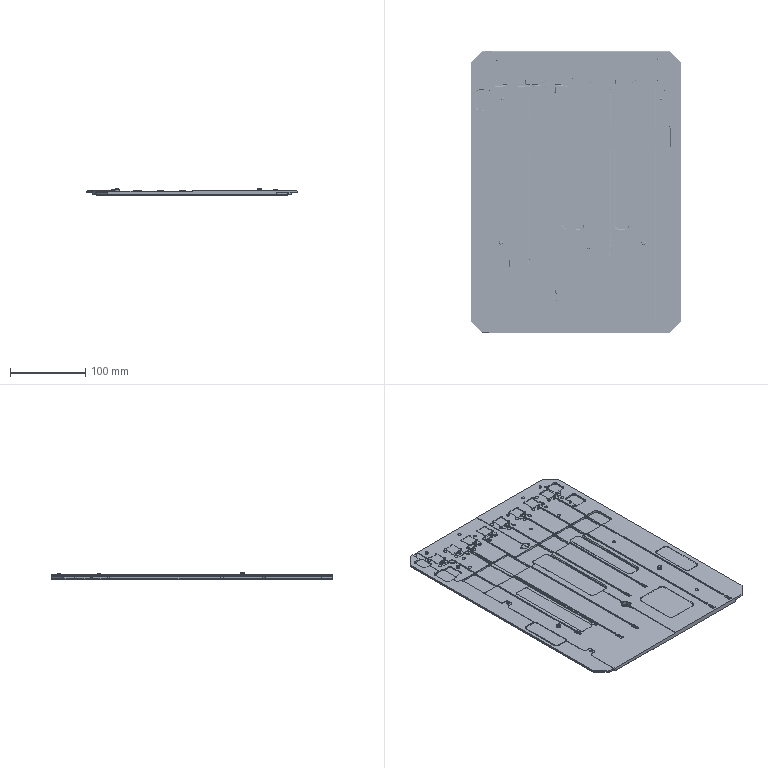CAM job | Mastercam | mm | 58 operations | part box 290 x 382 x 9.09
1. Facing | 1 - 80 面铣
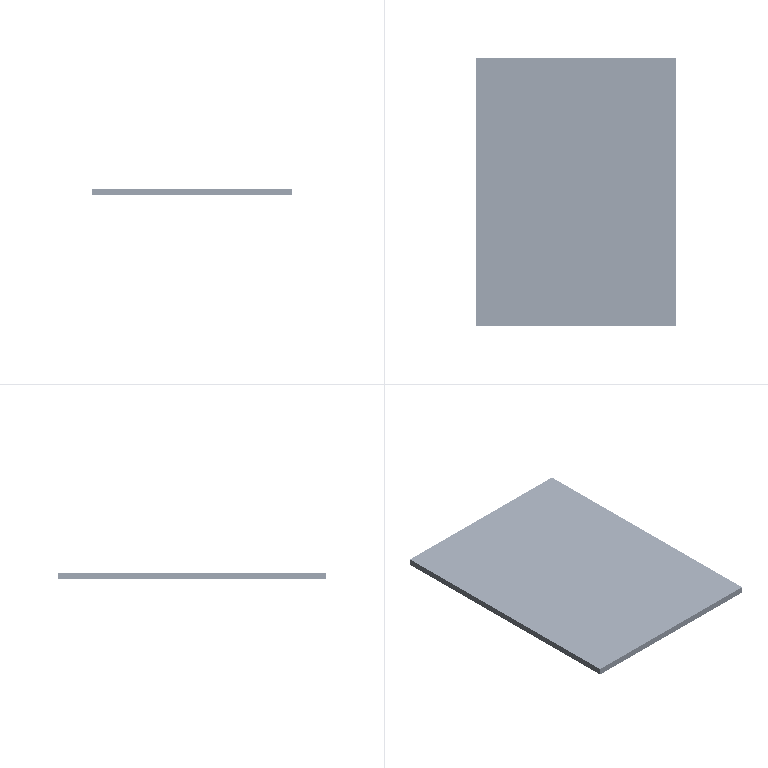2. Facing | 1 - 80 面铣
3. Contour (Ramp) | 9 - 10C 平底刀
4. Contour (2D) | 9 - 10C 平底刀
5. Contour (Ramp) | 6 - 6 平底刀
6. Contour (Remachining) | 22 - 3 平铣刀
7. Contour (Remachining) | 17 - 2 平铣刀
8. Drill/Counterbore | 2 - 4定位倒角
9. Peck Drill | 14 - 2.5 钻头
10. Peck Drill | 13 - 1.2 钻头
11. Peck Drill | 18 - 1.5 钻头
12. Peck Drill | 19 - 2 钻头
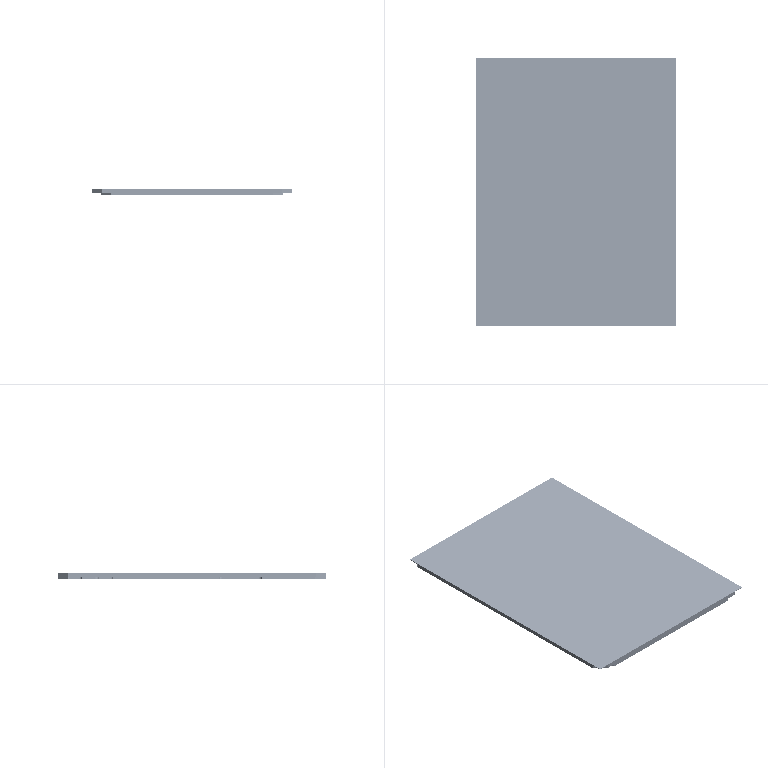13. Helix Bore | 22 - 3 平铣刀
14. Helix Bore | 22 - 3 平铣刀
15. Helix Bore | 6 - 6 平底刀
16. Surface Rough Pocket | 4 - 2-R0.5 圆鼻铣刀
17. 3D High Speed (Waterline) | 4 - 2-R0.5 圆鼻铣刀
18. Contour (Ramp) | 17 - 2 平铣刀
19. Contour (2D) | 17 - 2 平铣刀
20. Contour (Remachining) | 21 - 1 平铣刀
21. Contour (2D) | 10 - 10J 平底刀
22. Contour (2D) | 10 - 10J 平底刀
23. Contour (2D) | 22 - 3 平铣刀
24. Model Chamfer | 2 - 4定位倒角
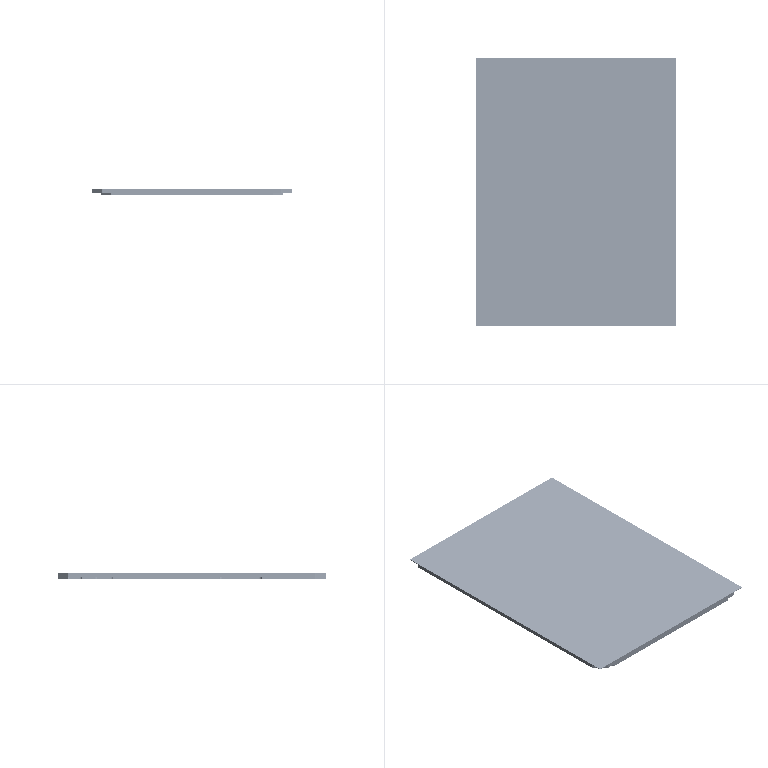25. Model Chamfer | 2 - 4定位倒角
26. Model Chamfer | 2 - 4定位倒角
27. Chamfer Drill | 2 - 4定位倒角
28. Circle Mill | 6 - 6 平底刀
29. Contour (Ramp) | 9 - 10C 平底刀
30. Surface Rough Pocket | 9 - 10C 平底刀
31. 挖槽策略 下午 09:55 | 6 - 6 平底刀
32. 挖槽策略 下午 09:55 | 7 - 4 平底刀
33. 3D High Speed (Waterline) | 6 - 6 平底刀
34. 3D High Speed (Horizontal) | 6 - 6 平底刀
35. Contour (2D) | 7 - 4 平底刀
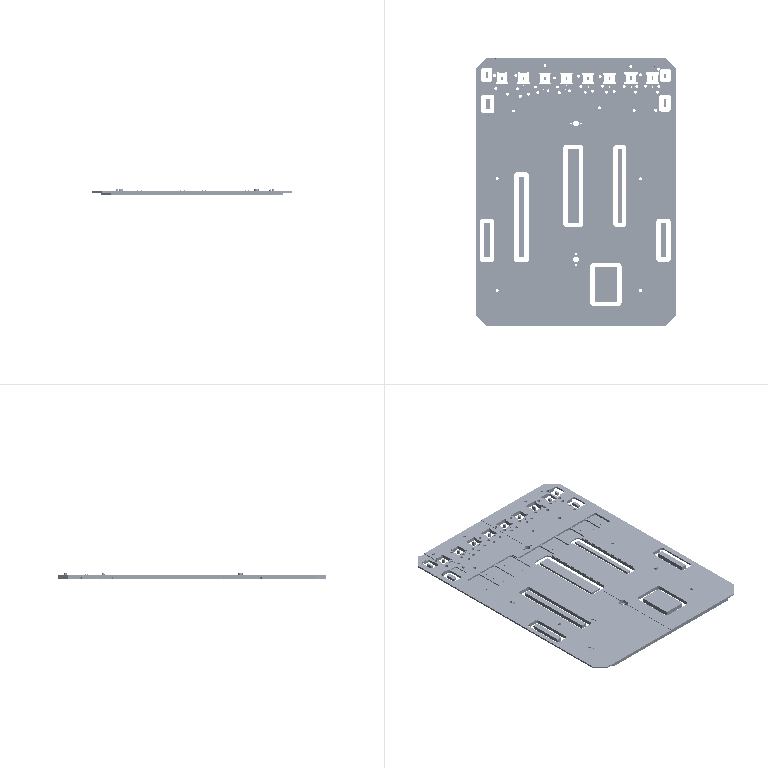36. Helix Bore | 6 - 6 平底刀
37. Circle Mill | 6 - 6 平底刀
38. Contour (Ramp) | 22 - 3 平铣刀
39. Contour (Remachining) | 17 - 2 平铣刀
40. Contour (2D) | 22 - 3 平铣刀
41. 3D High Speed (Waterline) | 4 - 2-R0.5 圆鼻铣刀
42. 挖槽策略 下午 09:55 | 22 - 3 平铣刀
43. 挖槽策略 下午 09:55 | 20 - 1.5 平铣刀
44. 挖槽策略 下午 09:55 | 21 - 1 平铣刀
45. 3D High Speed (Waterline) | 21 - 1 平铣刀
46. Contour (Ramp) | 23 - 0.5 平铣刀
47. Contour (Ramp) | 23 - 0.5 平铣刀
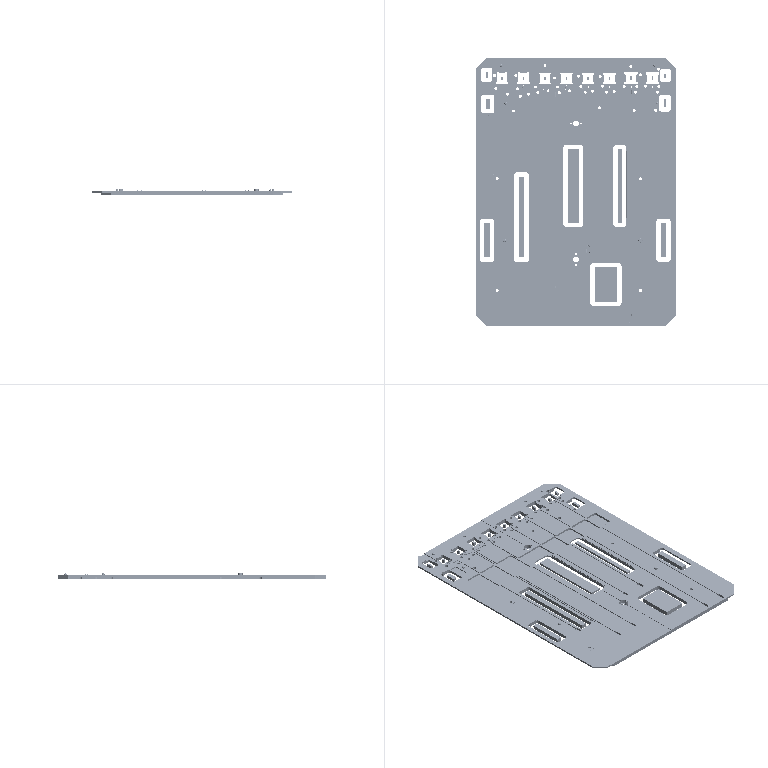48. Contour (Ramp) | 23 - 0.5 平铣刀
49. 3D High Speed (Waterline) | 23 - 0.5 平铣刀
50. Contour (2D) | 21 - 1 平铣刀
51. Contour (2D) | 21 - 1 平铣刀
52. Model Chamfer | 2 - 4定位倒角
53. Model Chamfer | 2 - 4定位倒角
54. Model Chamfer | 2 - 4定位倒角
55. Model Chamfer | 2 - 4定位倒角
56. Model Chamfer | 2 - 4定位倒角
57. Contour (2D chamfer) | 2 - 4定位倒角
58. Contour (2D) | 7 - 4 平底刀